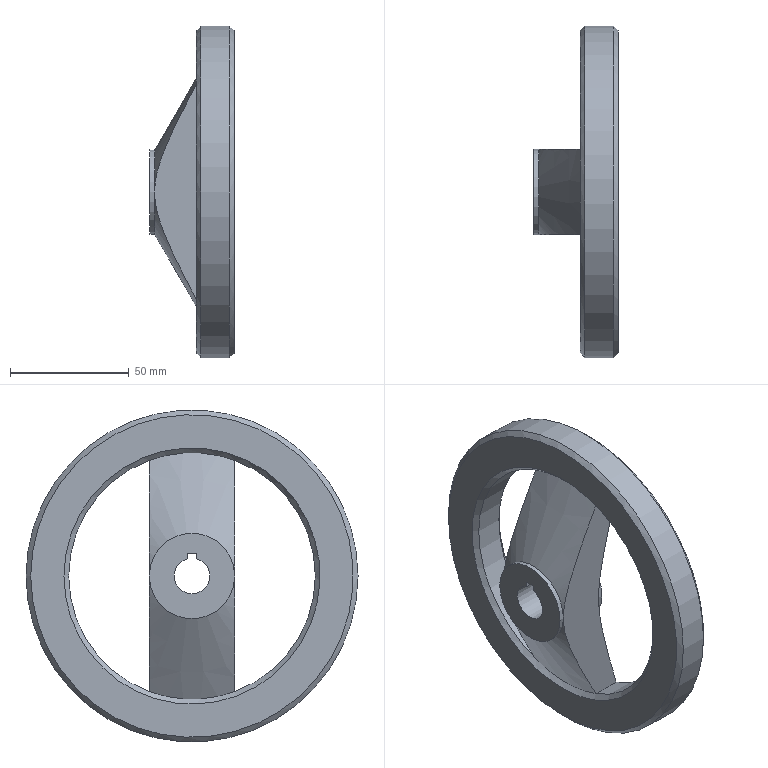Component | NX | HANDLE | 1 solid | 23 faces | volume 172274 mm3 | plane 9 | cone 8 | cylinder 6 | commonest cylinder face diameters 104 x2 36 x2 140 x1 15 x1